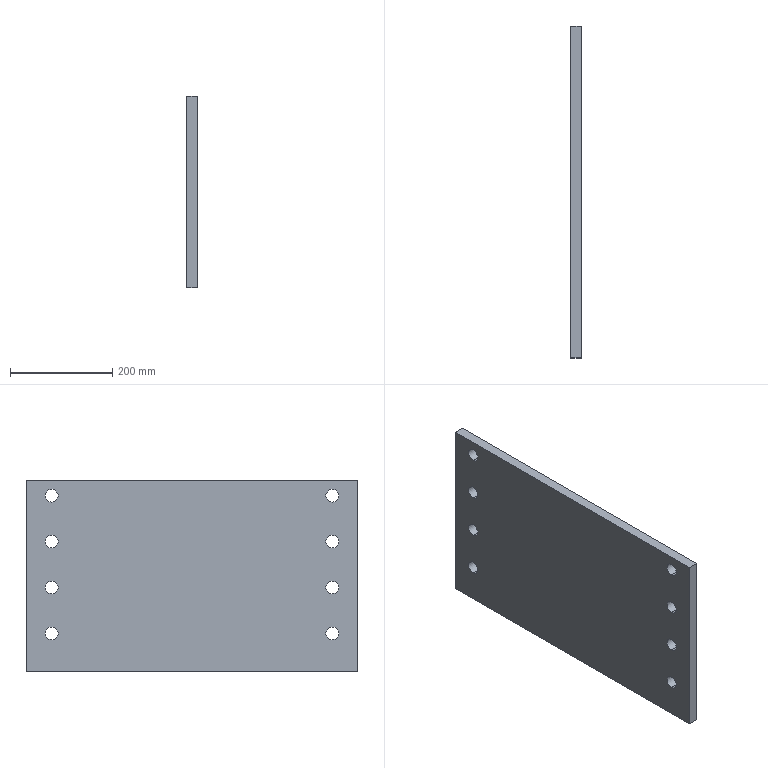Component | SolidWorks | Flange20-1 | 1 solid | 22 faces | box 20 x 650 x 375 mm | volume 4796460 mm3 | cylinder 16 | plane 6 | commonest cylinder face diameters 25 x16 | material Plain Carbon Steel
STEP:
#1=CARTESIAN_POINT('',(-121.74,86.469,201.908));
#2=VERTEX_POINT('',#1);
#3=CARTESIAN_POINT('',(-121.74,86.469,202.893));
#4=VERTEX_POINT('',#3);
#5=CARTESIAN_POINT('',(-121.74,86.469,202.401));
#6=DIRECTION('',(-1.,-0.,0.));
#7=DIRECTION('',(0.,0.,1.));
#8=AXIS2_PLACEMENT_3D('',#5,#6,#7);
#9=CIRCLE('',#8,0.4921);
#10=EDGE_CURVE('',#2,#4,#9,.T.);
#11=ORIENTED_EDGE('',*,*,#10,.F.);
#12=CARTESIAN_POINT('',(-122.528,86.469,201.908));
#13=VERTEX_POINT('',#12);
#14=CARTESIAN_POINT('',(-109.929,86.469,201.908));
#15=DIRECTION('',(-1.,-0.,0.));
#16=VECTOR('',#15,39.37);
#17=LINE('',#14,#16);
#18=EDGE_CURVE('',#2,#13,#17,.T.);
#19=ORIENTED_EDGE('',*,*,#18,.T.);
#20=CARTESIAN_POINT('',(-122.528,86.469,202.893));
#21=VERTEX_POINT('',#20);
#22=CARTESIAN_POINT('',(-122.528,86.469,202.401));
#23=DIRECTION('',(-1.,-0.,0.));
#24=DIRECTION('',(0.,0.,1.));
#25=AXIS2_PLACEMENT_3D('',#22,#23,#24);
#26=CIRCLE('',#25,0.4921);
#27=EDGE_CURVE('',#13,#21,#26,.T.);
#28=ORIENTED_EDGE('',*,*,#27,.T.);
#29=CARTESIAN_POINT('',(-109.929,86.469,202.893));
#30=DIRECTION('',(-1.,-0.,0.));
#31=VECTOR('',#30,39.37);
#32=LINE('',#29,#31);
#33=EDGE_CURVE('',#4,#21,#32,.T.);
#34=ORIENTED_EDGE('',*,*,#33,.F.);
#35=EDGE_LOOP('',(#11,#19,#28,#34));
#36=FACE_OUTER_BOUND('',#35,.T.);
#37=CARTESIAN_POINT('',(-109.929,86.469,202.401));
#38=DIRECTION('',(-1.,-0.,0.));
#39=DIRECTION('',(0.,0.,1.));
#40=AXIS2_PLACEMENT_3D('',#37,#38,#39);
#41=CYLINDRICAL_SURFACE('',#40,0.4921);
#42=ADVANCED_FACE('',(#36),#41,.F.);
#43=CARTESIAN_POINT('',(-121.74,86.469,198.365));
#44=VERTEX_POINT('',#43);
#45=CARTESIAN_POINT('',(-121.74,86.469,199.349));
#46=VERTEX_POINT('',#45);
#47=CARTESIAN_POINT('',(-121.74,86.469,198.857));
#48=DIRECTION('',(-1.,-0.,0.));
#49=DIRECTION('',(0.,0.,1.));
#50=AXIS2_PLACEMENT_3D('',#47,#48,#49);
#51=CIRCLE('',#50,0.4921);
#52=EDGE_CURVE('',#44,#46,#51,.T.);
#53=ORIENTED_EDGE('',*,*,#52,.F.);
#54=CARTESIAN_POINT('',(-122.528,86.469,198.365));
#55=VERTEX_POINT('',#54);
#56=CARTESIAN_POINT('',(-109.929,86.469,198.365));
#57=DIRECTION('',(-1.,-0.,0.));
#58=VECTOR('',#57,39.37);
#59=LINE('',#56,#58);
#60=EDGE_CURVE('',#44,#55,#59,.T.);
#61=ORIENTED_EDGE('',*,*,#60,.T.);
#62=CARTESIAN_POINT('',(-122.528,86.469,199.349));
#63=VERTEX_POINT('',#62);
#64=CARTESIAN_POINT('',(-122.528,86.469,198.857));
#65=DIRECTION('',(-1.,-0.,0.));
#66=DIRECTION('',(0.,0.,1.));
#67=AXIS2_PLACEMENT_3D('',#64,#65,#66);
#68=CIRCLE('',#67,0.4921);
#69=EDGE_CURVE('',#55,#63,#68,.T.);
#70=ORIENTED_EDGE('',*,*,#69,.T.);
#71=CARTESIAN_POINT('',(-109.929,86.469,199.349));
#72=DIRECTION('',(-1.,-0.,0.));
#73=VECTOR('',#72,39.37);
#74=LINE('',#71,#73);
#75=EDGE_CURVE('',#46,#63,#74,.T.);
#76=ORIENTED_EDGE('',*,*,#75,.F.);
#77=EDGE_LOOP('',(#53,#61,#70,#76));
#78=FACE_OUTER_BOUND('',#77,.T.);
#79=CARTESIAN_POINT('',(-109.929,86.469,198.857));
#80=DIRECTION('',(-1.,-0.,0.));
#81=DIRECTION('',(0.,0.,1.));
#82=AXIS2_PLACEMENT_3D('',#79,#80,#81);
#83=CYLINDRICAL_SURFACE('',#82,0.4921);
#84=ADVANCED_FACE('',(#78),#83,.F.);
#85=CARTESIAN_POINT('',(-121.74,86.469,194.822));
#86=VERTEX_POINT('',#85);
#87=CARTESIAN_POINT('',(-121.74,86.469,195.806));
#88=VERTEX_POINT('',#87);
#89=CARTESIAN_POINT('',(-121.74,86.469,195.314));
#90=DIRECTION('',(-1.,-0.,0.));
#91=DIRECTION('',(0.,0.,1.));
#92=AXIS2_PLACEMENT_3D('',#89,#90,#91);
#93=CIRCLE('',#92,0.4921);
#94=EDGE_CURVE('',#86,#88,#93,.T.);
#95=ORIENTED_EDGE('',*,*,#94,.F.);
#96=CARTESIAN_POINT('',(-122.528,86.469,194.822));
#97=VERTEX_POINT('',#96);
#98=CARTESIAN_POINT('',(-109.929,86.469,194.822));
#99=DIRECTION('',(-1.,-0.,0.));
#100=VECTOR('',#99,39.37);
#101=LINE('',#98,#100);
#102=EDGE_CURVE('',#86,#97,#101,.T.);
#103=ORIENTED_EDGE('',*,*,#102,.T.);
#104=CARTESIAN_POINT('',(-122.528,86.469,195.806));
#105=VERTEX_POINT('',#104);
#106=CARTESIAN_POINT('',(-122.528,86.469,195.314));
#107=DIRECTION('',(-1.,-0.,0.));
#108=DIRECTION('',(0.,0.,1.));
#109=AXIS2_PLACEMENT_3D('',#106,#107,#108);
#110=CIRCLE('',#109,0.4921);
#111=EDGE_CURVE('',#97,#105,#110,.T.);
#112=ORIENTED_EDGE('',*,*,#111,.T.);
#113=CARTESIAN_POINT('',(-109.929,86.469,195.806));
#114=DIRECTION('',(-1.,-0.,0.));
#115=VECTOR('',#114,39.37);
#116=LINE('',#113,#115);
#117=EDGE_CURVE('',#88,#105,#116,.T.);
#118=ORIENTED_EDGE('',*,*,#117,.F.);
#119=EDGE_LOOP('',(#95,#103,#112,#118));
#120=FACE_OUTER_BOUND('',#119,.T.);
#121=CARTESIAN_POINT('',(-109.929,86.469,195.314));
#122=DIRECTION('',(-1.,-0.,0.));
#123=DIRECTION('',(0.,0.,1.));
#124=AXIS2_PLACEMENT_3D('',#121,#122,#123);
#125=CYLINDRICAL_SURFACE('',#124,0.4921);
#126=ADVANCED_FACE('',(#120),#125,.F.);
#127=CARTESIAN_POINT('',(-121.74,64.816,194.822));
#128=VERTEX_POINT('',#127);
#129=CARTESIAN_POINT('',(-121.74,64.816,195.806));
#130=VERTEX_POINT('',#129);
#131=CARTESIAN_POINT('',(-121.74,64.816,195.314));
#132=DIRECTION('',(-1.,-0.,0.));
#133=DIRECTION('',(0.,0.,1.));
#134=AXIS2_PLACEMENT_3D('',#131,#132,#133);
#135=CIRCLE('',#134,0.4921);
#136=EDGE_CURVE('',#128,#130,#135,.T.);
#137=ORIENTED_EDGE('',*,*,#136,.F.);
#138=CARTESIAN_POINT('',(-122.528,64.816,194.822));
#139=VERTEX_POINT('',#138);
#140=CARTESIAN_POINT('',(-109.929,64.816,194.822));
#141=DIRECTION('',(-1.,-0.,0.));
#142=VECTOR('',#141,39.37);
#143=LINE('',#140,#142);
#144=EDGE_CURVE('',#128,#139,#143,.T.);
#145=ORIENTED_EDGE('',*,*,#144,.T.);
#146=CARTESIAN_POINT('',(-122.528,64.816,195.806));
#147=VERTEX_POINT('',#146);
#148=CARTESIAN_POINT('',(-122.528,64.816,195.314));
#149=DIRECTION('',(-1.,-0.,0.));
#150=DIRECTION('',(0.,0.,-1.));
#151=AXIS2_PLACEMENT_3D('',#148,#149,#150);
#152=CIRCLE('',#151,0.4921);
#153=EDGE_CURVE('',#139,#147,#152,.T.);
#154=ORIENTED_EDGE('',*,*,#153,.T.);
#155=CARTESIAN_POINT('',(-109.929,64.816,195.806));
#156=DIRECTION('',(-1.,-0.,0.));
#157=VECTOR('',#156,39.37);
#158=LINE('',#155,#157);
#159=EDGE_CURVE('',#130,#147,#158,.T.);
#160=ORIENTED_EDGE('',*,*,#159,.F.);
#161=EDGE_LOOP('',(#137,#145,#154,#160));
#162=FACE_OUTER_BOUND('',#161,.T.);
#163=CARTESIAN_POINT('',(-109.929,64.816,195.314));
#164=DIRECTION('',(-1.,-0.,0.));
#165=DIRECTION('',(0.,0.,1.));
#166=AXIS2_PLACEMENT_3D('',#163,#164,#165);
#167=CYLINDRICAL_SURFACE('',#166,0.4921);
#168=ADVANCED_FACE('',(#162),#167,.F.);
#169=CARTESIAN_POINT('',(-121.74,64.816,198.365));
#170=VERTEX_POINT('',#169);
#171=CARTESIAN_POINT('',(-121.74,64.816,199.349));
#172=VERTEX_POINT('',#171);
#173=CARTESIAN_POINT('',(-121.74,64.816,198.857));
#174=DIRECTION('',(-1.,-0.,0.));
#175=DIRECTION('',(0.,0.,1.));
#176=AXIS2_PLACEMENT_3D('',#173,#174,#175);
#177=CIRCLE('',#176,0.4921);
#178=EDGE_CURVE('',#170,#172,#177,.T.);
#179=ORIENTED_EDGE('',*,*,#178,.F.);
#180=CARTESIAN_POINT('',(-122.528,64.816,198.365));
#181=VERTEX_POINT('',#180);
#182=CARTESIAN_POINT('',(-109.929,64.816,198.365));
#183=DIRECTION('',(-1.,-0.,0.));
#184=VECTOR('',#183,39.37);
#185=LINE('',#182,#184);
#186=EDGE_CURVE('',#170,#181,#185,.T.);
#187=ORIENTED_EDGE('',*,*,#186,.T.);
#188=CARTESIAN_POINT('',(-122.528,64.816,199.349));
#189=VERTEX_POINT('',#188);
#190=CARTESIAN_POINT('',(-122.528,64.816,198.857));
#191=DIRECTION('',(-1.,-0.,0.));
#192=DIRECTION('',(0.,0.,-1.));
#193=AXIS2_PLACEMENT_3D('',#190,#191,#192);
#194=CIRCLE('',#193,0.4921);
#195=EDGE_CURVE('',#181,#189,#194,.T.);
#196=ORIENTED_EDGE('',*,*,#195,.T.);
#197=CARTESIAN_POINT('',(-109.929,64.816,199.349));
#198=DIRECTION('',(-1.,-0.,0.));
#199=VECTOR('',#198,39.37);
#200=LINE('',#197,#199);
#201=EDGE_CURVE('',#172,#189,#200,.T.);
#202=ORIENTED_EDGE('',*,*,#201,.F.);
#203=EDGE_LOOP('',(#179,#187,#196,#202));
#204=FACE_OUTER_BOUND('',#203,.T.);
#205=CARTESIAN_POINT('',(-109.929,64.816,198.857));
#206=DIRECTION('',(-1.,-0.,0.));
#207=DIRECTION('',(0.,0.,1.));
#208=AXIS2_PLACEMENT_3D('',#205,#206,#207);
#209=CYLINDRICAL_SURFACE('',#208,0.4921);
#210=ADVANCED_FACE('',(#204),#209,.F.);
#211=CARTESIAN_POINT('',(-121.74,64.816,201.908));
#212=VERTEX_POINT('',#211);
#213=CARTESIAN_POINT('',(-121.74,64.816,202.893));
#214=VERTEX_POINT('',#213);
#215=CARTESIAN_POINT('',(-121.74,64.816,202.401));
#216=DIRECTION('',(-1.,-0.,0.));
#217=DIRECTION('',(0.,0.,1.));
#218=AXIS2_PLACEMENT_3D('',#215,#216,#217);
#219=CIRCLE('',#218,0.4921);
#220=EDGE_CURVE('',#212,#214,#219,.T.);
#221=ORIENTED_EDGE('',*,*,#220,.F.);
#222=CARTESIAN_POINT('',(-122.528,64.816,201.908));
#223=VERTEX_POINT('',#222);
#224=CARTESIAN_POINT('',(-109.929,64.816,201.908));
#225=DIRECTION('',(-1.,-0.,0.));
#226=VECTOR('',#225,39.37);
#227=LINE('',#224,#226);
#228=EDGE_CURVE('',#212,#223,#227,.T.);
#229=ORIENTED_EDGE('',*,*,#228,.T.);
#230=CARTESIAN_POINT('',(-122.528,64.816,202.893));
#231=VERTEX_POINT('',#230);
#232=CARTESIAN_POINT('',(-122.528,64.816,202.401));
#233=DIRECTION('',(-1.,-0.,0.));
#234=DIRECTION('',(0.,0.,-1.));
#235=AXIS2_PLACEMENT_3D('',#232,#233,#234);
#236=CIRCLE('',#235,0.4921);
#237=EDGE_CURVE('',#223,#231,#236,.T.);
#238=ORIENTED_EDGE('',*,*,#237,.T.);
#239=CARTESIAN_POINT('',(-109.929,64.816,202.893));
#240=DIRECTION('',(-1.,-0.,0.));
#241=VECTOR('',#240,39.37);
#242=LINE('',#239,#241);
#243=EDGE_CURVE('',#214,#231,#242,.T.);
#244=ORIENTED_EDGE('',*,*,#243,.F.);
#245=EDGE_LOOP('',(#221,#229,#238,#244));
#246=FACE_OUTER_BOUND('',#245,.T.);
#247=CARTESIAN_POINT('',(-109.929,64.816,202.401));
#248=DIRECTION('',(-1.,-0.,0.));
#249=DIRECTION('',(0.,0.,1.));
#250=AXIS2_PLACEMENT_3D('',#247,#248,#249);
#251=CYLINDRICAL_SURFACE('',#250,0.4921);
#252=ADVANCED_FACE('',(#246),#251,.F.);
#253=CARTESIAN_POINT('',(-121.74,64.816,191.278));
#254=VERTEX_POINT('',#253);
#255=CARTESIAN_POINT('',(-121.74,64.816,192.263));
#256=VERTEX_POINT('',#255);
#257=CARTESIAN_POINT('',(-121.74,64.816,191.771));
#258=DIRECTION('',(-1.,-0.,0.));
#259=DIRECTION('',(0.,0.,1.));
#260=AXIS2_PLACEMENT_3D('',#257,#258,#259);
#261=CIRCLE('',#260,0.4921);
#262=EDGE_CURVE('',#254,#256,#261,.T.);
#263=ORIENTED_EDGE('',*,*,#262,.F.);
#264=CARTESIAN_POINT('',(-122.528,64.816,191.278));
#265=VERTEX_POINT('',#264);
#266=CARTESIAN_POINT('',(-109.929,64.816,191.278));
#267=DIRECTION('',(-1.,-0.,0.));
#268=VECTOR('',#267,39.37);
#269=LINE('',#266,#268);
#270=EDGE_CURVE('',#254,#265,#269,.T.);
#271=ORIENTED_EDGE('',*,*,#270,.T.);
#272=CARTESIAN_POINT('',(-122.528,64.816,192.263));
#273=VERTEX_POINT('',#272);
#274=CARTESIAN_POINT('',(-122.528,64.816,191.771));
#275=DIRECTION('',(-1.,-0.,0.));
#276=DIRECTION('',(0.,0.,-1.));
#277=AXIS2_PLACEMENT_3D('',#274,#275,#276);
#278=CIRCLE('',#277,0.4921);
#279=EDGE_CURVE('',#265,#273,#278,.T.);
#280=ORIENTED_EDGE('',*,*,#279,.T.);
#281=CARTESIAN_POINT('',(-109.929,64.816,192.263));
#282=DIRECTION('',(-1.,-0.,0.));
#283=VECTOR('',#282,39.37);
#284=LINE('',#281,#283);
#285=EDGE_CURVE('',#256,#273,#284,.T.);
#286=ORIENTED_EDGE('',*,*,#285,.F.);
#287=EDGE_LOOP('',(#263,#271,#280,#286));
#288=FACE_OUTER_BOUND('',#287,.T.);
#289=CARTESIAN_POINT('',(-109.929,64.816,191.771));
#290=DIRECTION('',(-1.,-0.,0.));
#291=DIRECTION('',(0.,0.,1.));
#292=AXIS2_PLACEMENT_3D('',#289,#290,#291);
#293=CYLINDRICAL_SURFACE('',#292,0.4921);
#294=ADVANCED_FACE('',(#288),#293,.F.);
#295=CARTESIAN_POINT('',(-121.74,86.469,191.278));
#296=VERTEX_POINT('',#295);
#297=CARTESIAN_POINT('',(-121.74,86.469,192.263));
#298=VERTEX_POINT('',#297);
#299=CARTESIAN_POINT('',(-121.74,86.469,191.771));
#300=DIRECTION('',(-1.,-0.,0.));
#301=DIRECTION('',(0.,0.,1.));
#302=AXIS2_PLACEMENT_3D('',#299,#300,#301);
#303=CIRCLE('',#302,0.4921);
#304=EDGE_CURVE('',#296,#298,#303,.T.);
#305=ORIENTED_EDGE('',*,*,#304,.F.);
#306=CARTESIAN_POINT('',(-122.528,86.469,191.278));
#307=VERTEX_POINT('',#306);
#308=CARTESIAN_POINT('',(-109.929,86.469,191.278));
#309=DIRECTION('',(-1.,-0.,0.));
#310=VECTOR('',#309,39.37);
#311=LINE('',#308,#310);
#312=EDGE_CURVE('',#296,#307,#311,.T.);
#313=ORIENTED_EDGE('',*,*,#312,.T.);
#314=CARTESIAN_POINT('',(-122.528,86.469,192.263));
#315=VERTEX_POINT('',#314);
#316=CARTESIAN_POINT('',(-122.528,86.469,191.771));
#317=DIRECTION('',(-1.,-0.,0.));
#318=DIRECTION('',(0.,0.,1.));
#319=AXIS2_PLACEMENT_3D('',#316,#317,#318);
#320=CIRCLE('',#319,0.4921);
#321=EDGE_CURVE('',#307,#315,#320,.T.);
#322=ORIENTED_EDGE('',*,*,#321,.T.);
#323=CARTESIAN_POINT('',(-109.929,86.469,192.263));
#324=DIRECTION('',(-1.,-0.,0.));
#325=VECTOR('',#324,39.37);
#326=LINE('',#323,#325);
#327=EDGE_CURVE('',#298,#315,#326,.T.);
#328=ORIENTED_EDGE('',*,*,#327,.F.);
#329=EDGE_LOOP('',(#305,#313,#322,#328));
#330=FACE_OUTER_BOUND('',#329,.T.);
#331=CARTESIAN_POINT('',(-109.929,86.469,191.771));
#332=DIRECTION('',(-1.,-0.,0.));
#333=DIRECTION('',(0.,0.,1.));
#334=AXIS2_PLACEMENT_3D('',#331,#332,#333);
#335=CYLINDRICAL_SURFACE('',#334,0.4921);
#336=ADVANCED_FACE('',(#330),#335,.F.);
#337=CARTESIAN_POINT('',(-122.528,88.438,203.582));
#338=VERTEX_POINT('',#337);
#339=CARTESIAN_POINT('',(-122.528,88.438,188.818));
#340=VERTEX_POINT('',#339);
#341=CARTESIAN_POINT('',(-122.528,88.438,205.353));
#342=DIRECTION('',(-0.,-0.,-1.));
#343=VECTOR('',#342,39.37);
#344=LINE('',#341,#343);
#345=EDGE_CURVE('',#338,#340,#344,.T.);
#346=ORIENTED_EDGE('',*,*,#345,.F.);
#347=CARTESIAN_POINT('',(-121.74,88.438,203.582));
#348=VERTEX_POINT('',#347);
#349=CARTESIAN_POINT('',(-122.528,88.438,203.582));
#350=DIRECTION('',(1.,0.,-0.));
#351=VECTOR('',#350,39.37);
#352=LINE('',#349,#351);
#353=EDGE_CURVE('',#338,#348,#352,.T.);
#354=ORIENTED_EDGE('',*,*,#353,.T.);
#355=CARTESIAN_POINT('',(-121.74,88.438,188.818));
#356=VERTEX_POINT('',#355);
#357=CARTESIAN_POINT('',(-121.74,88.438,205.353));
#358=DIRECTION('',(-0.,-0.,-1.));
#359=VECTOR('',#358,39.37);
#360=LINE('',#357,#359);
#361=EDGE_CURVE('',#348,#356,#360,.T.);
#362=ORIENTED_EDGE('',*,*,#361,.T.);
#363=CARTESIAN_POINT('',(-122.528,88.438,188.818));
#364=DIRECTION('',(1.,0.,-0.));
#365=VECTOR('',#364,39.37);
#366=LINE('',#363,#365);
#367=EDGE_CURVE('',#340,#356,#366,.T.);
#368=ORIENTED_EDGE('',*,*,#367,.F.);
#369=EDGE_LOOP('',(#346,#354,#362,#368));
#370=FACE_OUTER_BOUND('',#369,.T.);
#371=CARTESIAN_POINT('',(-120.756,88.438,204.566));
#372=DIRECTION('',(-0.,1.,-0.));
#373=DIRECTION('',(-1.,-0.,0.));
#374=AXIS2_PLACEMENT_3D('',#371,#372,#373);
#375=PLANE('',#374);
#376=ADVANCED_FACE('',(#370),#375,.T.);
#377=CARTESIAN_POINT('',(-121.74,86.469,202.401));
#378=DIRECTION('',(-1.,-0.,0.));
#379=DIRECTION('',(0.,0.,1.));
#380=AXIS2_PLACEMENT_3D('',#377,#378,#379);
#381=CIRCLE('',#380,0.4921);
#382=EDGE_CURVE('',#4,#2,#381,.T.);
#383=ORIENTED_EDGE('',*,*,#382,.T.);
#384=ORIENTED_EDGE('',*,*,#10,.T.);
#385=EDGE_LOOP('',(#383,#384));
#386=FACE_BOUND('',#385,.T.);
#387=CARTESIAN_POINT('',(-121.74,86.469,198.857));
#388=DIRECTION('',(-1.,-0.,0.));
#389=DIRECTION('',(0.,0.,1.));
#390=AXIS2_PLACEMENT_3D('',#387,#388,#389);
#391=CIRCLE('',#390,0.4921);
#392=EDGE_CURVE('',#46,#44,#391,.T.);
#393=ORIENTED_EDGE('',*,*,#392,.T.);
#394=ORIENTED_EDGE('',*,*,#52,.T.);
#395=EDGE_LOOP('',(#393,#394));
#396=FACE_BOUND('',#395,.T.);
#397=CARTESIAN_POINT('',(-121.74,86.469,195.314));
#398=DIRECTION('',(-1.,-0.,0.));
#399=DIRECTION('',(0.,0.,1.));
#400=AXIS2_PLACEMENT_3D('',#397,#398,#399);
#401=CIRCLE('',#400,0.4921);
#402=EDGE_CURVE('',#88,#86,#401,.T.);
#403=ORIENTED_EDGE('',*,*,#402,.T.);
#404=ORIENTED_EDGE('',*,*,#94,.T.);
#405=EDGE_LOOP('',(#403,#404));
#406=FACE_BOUND('',#405,.T.);
#407=CARTESIAN_POINT('',(-121.74,64.816,195.314));
#408=DIRECTION('',(-1.,-0.,0.));
#409=DIRECTION('',(0.,0.,1.));
#410=AXIS2_PLACEMENT_3D('',#407,#408,#409);
#411=CIRCLE('',#410,0.4921);
#412=EDGE_CURVE('',#130,#128,#411,.T.);
#413=ORIENTED_EDGE('',*,*,#412,.T.);
#414=ORIENTED_EDGE('',*,*,#136,.T.);
#415=EDGE_LOOP('',(#413,#414));
#416=FACE_BOUND('',#415,.T.);
#417=CARTESIAN_POINT('',(-121.74,64.816,198.857));
#418=DIRECTION('',(-1.,-0.,0.));
#419=DIRECTION('',(0.,0.,1.));
#420=AXIS2_PLACEMENT_3D('',#417,#418,#419);
#421=CIRCLE('',#420,0.4921);
#422=EDGE_CURVE('',#172,#170,#421,.T.);
#423=ORIENTED_EDGE('',*,*,#422,.T.);
#424=ORIENTED_EDGE('',*,*,#178,.T.);
#425=EDGE_LOOP('',(#423,#424));
#426=FACE_BOUND('',#425,.T.);
#427=CARTESIAN_POINT('',(-121.74,64.816,202.401));
#428=DIRECTION('',(-1.,-0.,0.));
#429=DIRECTION('',(0.,0.,1.));
#430=AXIS2_PLACEMENT_3D('',#427,#428,#429);
#431=CIRCLE('',#430,0.4921);
#432=EDGE_CURVE('',#214,#212,#431,.T.);
#433=ORIENTED_EDGE('',*,*,#432,.T.);
#434=ORIENTED_EDGE('',*,*,#220,.T.);
#435=EDGE_LOOP('',(#433,#434));
#436=FACE_BOUND('',#435,.T.);
#437=CARTESIAN_POINT('',(-121.74,64.816,191.771));
#438=DIRECTION('',(-1.,-0.,0.));
#439=DIRECTION('',(0.,0.,1.));
#440=AXIS2_PLACEMENT_3D('',#437,#438,#439);
#441=CIRCLE('',#440,0.4921);
#442=EDGE_CURVE('',#256,#254,#441,.T.);
#443=ORIENTED_EDGE('',*,*,#442,.T.);
#444=ORIENTED_EDGE('',*,*,#262,.T.);
#445=EDGE_LOOP('',(#443,#444));
#446=FACE_BOUND('',#445,.T.);
#447=CARTESIAN_POINT('',(-121.74,86.469,191.771));
#448=DIRECTION('',(-1.,-0.,0.));
#449=DIRECTION('',(0.,0.,1.));
#450=AXIS2_PLACEMENT_3D('',#447,#448,#449);
#451=CIRCLE('',#450,0.4921);
#452=EDGE_CURVE('',#298,#296,#451,.T.);
#453=ORIENTED_EDGE('',*,*,#452,.T.);
#454=ORIENTED_EDGE('',*,*,#304,.T.);
#455=EDGE_LOOP('',(#453,#454));
#456=FACE_BOUND('',#455,.T.);
#457=CARTESIAN_POINT('',(-121.74,62.847,203.582));
#458=VERTEX_POINT('',#457);
#459=CARTESIAN_POINT('',(-121.74,62.847,188.818));
#460=VERTEX_POINT('',#459);
#461=CARTESIAN_POINT('',(-121.74,62.847,205.353));
#462=DIRECTION('',(-0.,-0.,-1.));
#463=VECTOR('',#462,39.37);
#464=LINE('',#461,#463);
#465=EDGE_CURVE('',#458,#460,#464,.T.);
#466=ORIENTED_EDGE('',*,*,#465,.T.);
#467=CARTESIAN_POINT('',(-121.74,88.438,188.818));
#468=DIRECTION('',(0.,-1.,0.));
#469=VECTOR('',#468,39.37);
#470=LINE('',#467,#469);
#471=EDGE_CURVE('',#356,#460,#470,.T.);
#472=ORIENTED_EDGE('',*,*,#471,.F.);
#473=ORIENTED_EDGE('',*,*,#361,.F.);
#474=CARTESIAN_POINT('',(-121.74,88.438,203.582));
#475=DIRECTION('',(0.,-1.,0.));
#476=VECTOR('',#475,39.37);
#477=LINE('',#474,#476);
#478=EDGE_CURVE('',#348,#458,#477,.T.);
#479=ORIENTED_EDGE('',*,*,#478,.T.);
#480=EDGE_LOOP('',(#466,#472,#473,#479));
#481=FACE_OUTER_BOUND('',#480,.T.);
#482=CARTESIAN_POINT('',(-121.74,88.438,205.353));
#483=DIRECTION('',(-1.,-0.,0.));
#484=DIRECTION('',(0.,0.,1.));
#485=AXIS2_PLACEMENT_3D('',#482,#483,#484);
#486=PLANE('',#485);
#487=ADVANCED_FACE('',(#386,#396,#406,#416,#426,#436,#446,#456,#481),#486,.F.);
#488=CARTESIAN_POINT('',(-122.528,62.847,188.818));
#489=VERTEX_POINT('',#488);
#490=CARTESIAN_POINT('',(-122.528,62.847,188.818));
#491=DIRECTION('',(1.,0.,-0.));
#492=VECTOR('',#491,39.37);
#493=LINE('',#490,#492);
#494=EDGE_CURVE('',#489,#460,#493,.T.);
#495=ORIENTED_EDGE('',*,*,#494,.F.);
#496=CARTESIAN_POINT('',(-122.528,88.438,188.818));
#497=DIRECTION('',(0.,-1.,0.));
#498=VECTOR('',#497,39.37);
#499=LINE('',#496,#498);
#500=EDGE_CURVE('',#340,#489,#499,.T.);
#501=ORIENTED_EDGE('',*,*,#500,.F.);
#502=ORIENTED_EDGE('',*,*,#367,.T.);
#503=ORIENTED_EDGE('',*,*,#471,.T.);
#504=EDGE_LOOP('',(#495,#501,#502,#503));
#505=FACE_OUTER_BOUND('',#504,.T.);
#506=CARTESIAN_POINT('',(-122.528,88.438,188.818));
#507=DIRECTION('',(-0.,-0.,-1.));
#508=DIRECTION('',(-1.,-0.,0.));
#509=AXIS2_PLACEMENT_3D('',#506,#507,#508);
#510=PLANE('',#509);
#511=ADVANCED_FACE('',(#505),#510,.T.);
#512=CARTESIAN_POINT('',(-122.528,86.469,202.401));
#513=DIRECTION('',(-1.,-0.,0.));
#514=DIRECTION('',(0.,0.,1.));
#515=AXIS2_PLACEMENT_3D('',#512,#513,#514);
#516=CIRCLE('',#515,0.4921);
#517=EDGE_CURVE('',#21,#13,#516,.T.);
#518=ORIENTED_EDGE('',*,*,#517,.F.);
#519=ORIENTED_EDGE('',*,*,#27,.F.);
#520=EDGE_LOOP('',(#518,#519));
#521=FACE_BOUND('',#520,.T.);
#522=CARTESIAN_POINT('',(-122.528,86.469,198.857));
#523=DIRECTION('',(-1.,-0.,0.));
#524=DIRECTION('',(0.,0.,1.));
#525=AXIS2_PLACEMENT_3D('',#522,#523,#524);
#526=CIRCLE('',#525,0.4921);
#527=EDGE_CURVE('',#63,#55,#526,.T.);
#528=ORIENTED_EDGE('',*,*,#527,.F.);
#529=ORIENTED_EDGE('',*,*,#69,.F.);
#530=EDGE_LOOP('',(#528,#529));
#531=FACE_BOUND('',#530,.T.);
#532=CARTESIAN_POINT('',(-122.528,86.469,195.314));
#533=DIRECTION('',(-1.,-0.,0.));
#534=DIRECTION('',(0.,0.,1.));
#535=AXIS2_PLACEMENT_3D('',#532,#533,#534);
#536=CIRCLE('',#535,0.4921);
#537=EDGE_CURVE('',#105,#97,#536,.T.);
#538=ORIENTED_EDGE('',*,*,#537,.F.);
#539=ORIENTED_EDGE('',*,*,#111,.F.);
#540=EDGE_LOOP('',(#538,#539));
#541=FACE_BOUND('',#540,.T.);
#542=CARTESIAN_POINT('',(-122.528,64.816,195.314));
#543=DIRECTION('',(-1.,-0.,0.));
#544=DIRECTION('',(0.,0.,-1.));
#545=AXIS2_PLACEMENT_3D('',#542,#543,#544);
#546=CIRCLE('',#545,0.4921);
#547=EDGE_CURVE('',#147,#139,#546,.T.);
#548=ORIENTED_EDGE('',*,*,#547,.F.);
#549=ORIENTED_EDGE('',*,*,#153,.F.);
#550=EDGE_LOOP('',(#548,#549));
#551=FACE_BOUND('',#550,.T.);
#552=CARTESIAN_POINT('',(-122.528,64.816,198.857));
#553=DIRECTION('',(-1.,-0.,0.));
#554=DIRECTION('',(0.,0.,-1.));
#555=AXIS2_PLACEMENT_3D('',#552,#553,#554);
#556=CIRCLE('',#555,0.4921);
#557=EDGE_CURVE('',#189,#181,#556,.T.);
#558=ORIENTED_EDGE('',*,*,#557,.F.);
#559=ORIENTED_EDGE('',*,*,#195,.F.);
#560=EDGE_LOOP('',(#558,#559));
#561=FACE_BOUND('',#560,.T.);
#562=CARTESIAN_POINT('',(-122.528,64.816,202.401));
#563=DIRECTION('',(-1.,-0.,0.));
#564=DIRECTION('',(0.,0.,-1.));
#565=AXIS2_PLACEMENT_3D('',#562,#563,#564);
#566=CIRCLE('',#565,0.4921);
#567=EDGE_CURVE('',#231,#223,#566,.T.);
#568=ORIENTED_EDGE('',*,*,#567,.F.);
#569=ORIENTED_EDGE('',*,*,#237,.F.);
#570=EDGE_LOOP('',(#568,#569));
#571=FACE_BOUND('',#570,.T.);
#572=CARTESIAN_POINT('',(-122.528,64.816,191.771));
#573=DIRECTION('',(-1.,-0.,0.));
#574=DIRECTION('',(0.,0.,-1.));
#575=AXIS2_PLACEMENT_3D('',#572,#573,#574);
#576=CIRCLE('',#575,0.4921);
#577=EDGE_CURVE('',#273,#265,#576,.T.);
#578=ORIENTED_EDGE('',*,*,#577,.F.);
#579=ORIENTED_EDGE('',*,*,#279,.F.);
#580=EDGE_LOOP('',(#578,#579));
#581=FACE_BOUND('',#580,.T.);
#582=CARTESIAN_POINT('',(-122.528,86.469,191.771));
#583=DIRECTION('',(-1.,-0.,0.));
#584=DIRECTION('',(0.,0.,1.));
#585=AXIS2_PLACEMENT_3D('',#582,#583,#584);
#586=CIRCLE('',#585,0.4921);
#587=EDGE_CURVE('',#315,#307,#586,.T.);
#588=ORIENTED_EDGE('',*,*,#587,.F.);
#589=ORIENTED_EDGE('',*,*,#321,.F.);
#590=EDGE_LOOP('',(#588,#589));
#591=FACE_BOUND('',#590,.T.);
#592=CARTESIAN_POINT('',(-122.528,62.847,203.582));
#593=VERTEX_POINT('',#592);
#594=CARTESIAN_POINT('',(-122.528,62.847,205.353));
#595=DIRECTION('',(-0.,-0.,-1.));
#596=VECTOR('',#595,39.37);
#597=LINE('',#594,#596);
#598=EDGE_CURVE('',#593,#489,#597,.T.);
#599=ORIENTED_EDGE('',*,*,#598,.F.);
#600=CARTESIAN_POINT('',(-122.528,88.438,203.582));
#601=DIRECTION('',(0.,-1.,0.));
#602=VECTOR('',#601,39.37);
#603=LINE('',#600,#602);
#604=EDGE_CURVE('',#338,#593,#603,.T.);
#605=ORIENTED_EDGE('',*,*,#604,.F.);
#606=ORIENTED_EDGE('',*,*,#345,.T.);
#607=ORIENTED_EDGE('',*,*,#500,.T.);
#608=EDGE_LOOP('',(#599,#605,#606,#607));
#609=FACE_OUTER_BOUND('',#608,.T.);
#610=CARTESIAN_POINT('',(-122.528,88.438,205.353));
#611=DIRECTION('',(-1.,-0.,0.));
#612=DIRECTION('',(0.,0.,1.));
#613=AXIS2_PLACEMENT_3D('',#610,#611,#612);
#614=PLANE('',#613);
#615=ADVANCED_FACE('',(#521,#531,#541,#551,#561,#571,#581,#591,#609),#614,.T.);
#616=ORIENTED_EDGE('',*,*,#465,.F.);
#617=CARTESIAN_POINT('',(-121.74,62.847,203.582));
#618=DIRECTION('',(-1.,-0.,0.));
#619=VECTOR('',#618,39.37);
#620=LINE('',#617,#619);
#621=EDGE_CURVE('',#458,#593,#620,.T.);
#622=ORIENTED_EDGE('',*,*,#621,.T.);
#623=ORIENTED_EDGE('',*,*,#598,.T.);
#624=ORIENTED_EDGE('',*,*,#494,.T.);
#625=EDGE_LOOP('',(#616,#622,#623,#624));
#626=FACE_OUTER_BOUND('',#625,.T.);
#627=CARTESIAN_POINT('',(-120.756,62.847,203.582));
#628=DIRECTION('',(-0.,1.,-0.));
#629=DIRECTION('',(-1.,-0.,0.));
#630=AXIS2_PLACEMENT_3D('',#627,#628,#629);
#631=PLANE('',#630);
#632=ADVANCED_FACE('',(#626),#631,.F.);
#633=ORIENTED_EDGE('',*,*,#312,.F.);
#634=ORIENTED_EDGE('',*,*,#452,.F.);
#635=ORIENTED_EDGE('',*,*,#327,.T.);
#636=ORIENTED_EDGE('',*,*,#587,.T.);
#637=EDGE_LOOP('',(#633,#634,#635,#636));
#638=FACE_OUTER_BOUND('',#637,.T.);
#639=CARTESIAN_POINT('',(-109.929,86.469,191.771));
#640=DIRECTION('',(-1.,-0.,0.));
#641=DIRECTION('',(0.,0.,1.));
#642=AXIS2_PLACEMENT_3D('',#639,#640,#641);
#643=CYLINDRICAL_SURFACE('',#642,0.4921);
#644=ADVANCED_FACE('',(#638),#643,.F.);
#645=ORIENTED_EDGE('',*,*,#270,.F.);
#646=ORIENTED_EDGE('',*,*,#442,.F.);
#647=ORIENTED_EDGE('',*,*,#285,.T.);
#648=ORIENTED_EDGE('',*,*,#577,.T.);
#649=EDGE_LOOP('',(#645,#646,#647,#648));
#650=FACE_OUTER_BOUND('',#649,.T.);
#651=CARTESIAN_POINT('',(-109.929,64.816,191.771));
#652=DIRECTION('',(-1.,-0.,0.));
#653=DIRECTION('',(0.,0.,1.));
#654=AXIS2_PLACEMENT_3D('',#651,#652,#653);
#655=CYLINDRICAL_SURFACE('',#654,0.4921);
#656=ADVANCED_FACE('',(#650),#655,.F.);
#657=ORIENTED_EDGE('',*,*,#228,.F.);
#658=ORIENTED_EDGE('',*,*,#432,.F.);
#659=ORIENTED_EDGE('',*,*,#243,.T.);
#660=ORIENTED_EDGE('',*,*,#567,.T.);
#661=EDGE_LOOP('',(#657,#658,#659,#660));
#662=FACE_OUTER_BOUND('',#661,.T.);
#663=CARTESIAN_POINT('',(-109.929,64.816,202.401));
#664=DIRECTION('',(-1.,-0.,0.));
#665=DIRECTION('',(0.,0.,1.));
#666=AXIS2_PLACEMENT_3D('',#663,#664,#665);
#667=CYLINDRICAL_SURFACE('',#666,0.4921);
#668=ADVANCED_FACE('',(#662),#667,.F.);
#669=ORIENTED_EDGE('',*,*,#186,.F.);
#670=ORIENTED_EDGE('',*,*,#422,.F.);
#671=ORIENTED_EDGE('',*,*,#201,.T.);
#672=ORIENTED_EDGE('',*,*,#557,.T.);
#673=EDGE_LOOP('',(#669,#670,#671,#672));
#674=FACE_OUTER_BOUND('',#673,.T.);
#675=CARTESIAN_POINT('',(-109.929,64.816,198.857));
#676=DIRECTION('',(-1.,-0.,0.));
#677=DIRECTION('',(0.,0.,1.));
#678=AXIS2_PLACEMENT_3D('',#675,#676,#677);
#679=CYLINDRICAL_SURFACE('',#678,0.4921);
#680=ADVANCED_FACE('',(#674),#679,.F.);
#681=ORIENTED_EDGE('',*,*,#144,.F.);
#682=ORIENTED_EDGE('',*,*,#412,.F.);
#683=ORIENTED_EDGE('',*,*,#159,.T.);
#684=ORIENTED_EDGE('',*,*,#547,.T.);
#685=EDGE_LOOP('',(#681,#682,#683,#684));
#686=FACE_OUTER_BOUND('',#685,.T.);
#687=CARTESIAN_POINT('',(-109.929,64.816,195.314));
#688=DIRECTION('',(-1.,-0.,0.));
#689=DIRECTION('',(0.,0.,1.));
#690=AXIS2_PLACEMENT_3D('',#687,#688,#689);
#691=CYLINDRICAL_SURFACE('',#690,0.4921);
#692=ADVANCED_FACE('',(#686),#691,.F.);
#693=ORIENTED_EDGE('',*,*,#102,.F.);
#694=ORIENTED_EDGE('',*,*,#402,.F.);
#695=ORIENTED_EDGE('',*,*,#117,.T.);
#696=ORIENTED_EDGE('',*,*,#537,.T.);
#697=EDGE_LOOP('',(#693,#694,#695,#696));
#698=FACE_OUTER_BOUND('',#697,.T.);
#699=CARTESIAN_POINT('',(-109.929,86.469,195.314));
#700=DIRECTION('',(-1.,-0.,0.));
#701=DIRECTION('',(0.,0.,1.));
#702=AXIS2_PLACEMENT_3D('',#699,#700,#701);
#703=CYLINDRICAL_SURFACE('',#702,0.4921);
#704=ADVANCED_FACE('',(#698),#703,.F.);
#705=ORIENTED_EDGE('',*,*,#60,.F.);
#706=ORIENTED_EDGE('',*,*,#392,.F.);
#707=ORIENTED_EDGE('',*,*,#75,.T.);
#708=ORIENTED_EDGE('',*,*,#527,.T.);
#709=EDGE_LOOP('',(#705,#706,#707,#708));
#710=FACE_OUTER_BOUND('',#709,.T.);
#711=CARTESIAN_POINT('',(-109.929,86.469,198.857));
#712=DIRECTION('',(-1.,-0.,0.));
#713=DIRECTION('',(0.,0.,1.));
#714=AXIS2_PLACEMENT_3D('',#711,#712,#713);
#715=CYLINDRICAL_SURFACE('',#714,0.4921);
#716=ADVANCED_FACE('',(#710),#715,.F.);
#717=ORIENTED_EDGE('',*,*,#18,.F.);
#718=ORIENTED_EDGE('',*,*,#382,.F.);
#719=ORIENTED_EDGE('',*,*,#33,.T.);
#720=ORIENTED_EDGE('',*,*,#517,.T.);
#721=EDGE_LOOP('',(#717,#718,#719,#720));
#722=FACE_OUTER_BOUND('',#721,.T.);
#723=CARTESIAN_POINT('',(-109.929,86.469,202.401));
#724=DIRECTION('',(-1.,-0.,0.));
#725=DIRECTION('',(0.,0.,1.));
#726=AXIS2_PLACEMENT_3D('',#723,#724,#725);
#727=CYLINDRICAL_SURFACE('',#726,0.4921);
#728=ADVANCED_FACE('',(#722),#727,.F.);
#729=ORIENTED_EDGE('',*,*,#353,.F.);
#730=ORIENTED_EDGE('',*,*,#604,.T.);
#731=ORIENTED_EDGE('',*,*,#621,.F.);
#732=ORIENTED_EDGE('',*,*,#478,.F.);
#733=EDGE_LOOP('',(#729,#730,#731,#732));
#734=FACE_OUTER_BOUND('',#733,.T.);
#735=CARTESIAN_POINT('',(-109.929,88.438,203.582));
#736=DIRECTION('',(-0.,-0.,-1.));
#737=DIRECTION('',(-1.,-0.,0.));
#738=AXIS2_PLACEMENT_3D('',#735,#736,#737);
#739=PLANE('',#738);
#740=ADVANCED_FACE('',(#734),#739,.F.);
#741=CLOSED_SHELL('',(#42,#84,#126,#168,#210,#252,#294,#336,#376,#487,#511,#615,#632,#644,#656,#668,#680,#692,#704,#716,#728,#740));
#742=MANIFOLD_SOLID_BREP('',#741);
#743=CARTESIAN_POINT('',(0.,0.,0.));
#744=DIRECTION('',(0.,0.,1.));
#745=DIRECTION('',(1.,0.,0.));
#746=AXIS2_PLACEMENT_3D('',#743,#744,#745);
#747=(LENGTH_UNIT()NAMED_UNIT(*)SI_UNIT($,.METRE.));
#748=LENGTH_MEASURE_WITH_UNIT(LENGTH_MEASURE(0.0254),#747);
#749=DIMENSIONAL_EXPONENTS(1.,0.,0.,0.,0.,0.,0.);
#750=(CONVERSION_BASED_UNIT('',#748)LENGTH_UNIT()NAMED_UNIT(#749));
#751=UNCERTAINTY_MEASURE_WITH_UNIT(LENGTH_MEASURE(0.00001),#750,'','');
#752=(NAMED_UNIT(*)PLANE_ANGLE_UNIT()SI_UNIT($,.RADIAN.));
#753=(NAMED_UNIT(*)SI_UNIT($,.STERADIAN.)SOLID_ANGLE_UNIT());
#754=(GEOMETRIC_REPRESENTATION_CONTEXT(3)GLOBAL_UNCERTAINTY_ASSIGNED_CONTEXT((#751))GLOBAL_UNIT_ASSIGNED_CONTEXT((#750,#752,#753))REPRESENTATION_CONTEXT('',''));
#755=ADVANCED_BREP_SHAPE_REPRESENTATION('',(#742,#746),#754);
#756=COLOUR_RGB('',0.7922,0.8196,0.9333);
#757=FILL_AREA_STYLE_COLOUR('',#756);
#758=FILL_AREA_STYLE('',(#757));
#759=SURFACE_STYLE_FILL_AREA(#758);
#760=SURFACE_SIDE_STYLE('',(#759));
#761=SURFACE_STYLE_USAGE(.BOTH.,#760);
#762=PRESENTATION_STYLE_ASSIGNMENT((#761));
#763=STYLED_ITEM('',(#762),#742);
#764=(LENGTH_UNIT()NAMED_UNIT(*)SI_UNIT($,.METRE.));
#765=LENGTH_MEASURE_WITH_UNIT(LENGTH_MEASURE(0.0254),#764);
#766=DIMENSIONAL_EXPONENTS(1.,0.,0.,0.,0.,0.,0.);
#767=(CONVERSION_BASED_UNIT('',#765)LENGTH_UNIT()NAMED_UNIT(#766));
#768=UNCERTAINTY_MEASURE_WITH_UNIT(LENGTH_MEASURE(0.00001),#767,'','');
#769=(NAMED_UNIT(*)PLANE_ANGLE_UNIT()SI_UNIT($,.RADIAN.));
#770=(NAMED_UNIT(*)SI_UNIT($,.STERADIAN.)SOLID_ANGLE_UNIT());
#771=(GEOMETRIC_REPRESENTATION_CONTEXT(3)GLOBAL_UNCERTAINTY_ASSIGNED_CONTEXT((#768))GLOBAL_UNIT_ASSIGNED_CONTEXT((#767,#769,#770))REPRESENTATION_CONTEXT('',''));
#772=MECHANICAL_DESIGN_GEOMETRIC_PRESENTATION_REPRESENTATION('',(#763),#771);
#773=PRESENTATION_LAYER_ASSIGNMENT('','',(#763));